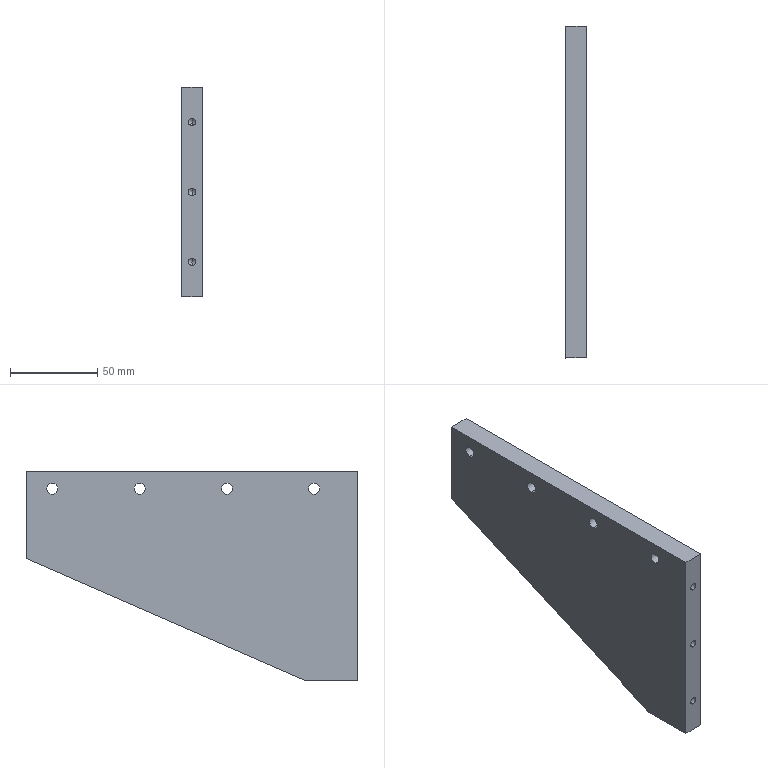Component | SolidWorks | V1ZHXTZ-AxisMountingPlateReinforcementPlateSB1-1 | 1 solid | 39 faces | box 12 x 190 x 120 mm | volume 202405 mm3 | cylinder 22 | plane 11 | cone 6 | commonest cylinder face diameters 11 x8 6.4 x8 4.2 x6
STEP:
#1=COLOUR_RGB('',0.7922,0.8196,0.9333);
#2=FILL_AREA_STYLE_COLOUR('',#1);
#3=FILL_AREA_STYLE('',(#2));
#4=SURFACE_STYLE_FILL_AREA(#3);
#5=SURFACE_SIDE_STYLE('',(#4));
#6=SURFACE_STYLE_USAGE(.BOTH.,#5);
#7=PRESENTATION_STYLE_ASSIGNMENT((#6));
#8=CARTESIAN_POINT('',(9.745,-12.863,21.687));
#9=VERTEX_POINT('',#8);
#10=CARTESIAN_POINT('',(9.745,-12.863,21.521));
#11=VERTEX_POINT('',#10);
#12=CARTESIAN_POINT('',(9.745,-12.863,21.604));
#13=DIRECTION('',(0.,-1.,-0.));
#14=DIRECTION('',(0.,0.,-1.));
#15=AXIS2_PLACEMENT_3D('',#12,#13,#14);
#16=CIRCLE('',#15,0.08268);
#17=EDGE_CURVE('',#9,#11,#16,.T.);
#18=ORIENTED_EDGE('',*,*,#17,.F.);
#19=CARTESIAN_POINT('',(9.745,-13.548,21.687));
#20=VERTEX_POINT('',#19);
#21=CARTESIAN_POINT('',(9.745,-13.548,21.687));
#22=DIRECTION('',(0.,-1.,-0.));
#23=VECTOR('',#22,39.37);
#24=LINE('',#21,#23);
#25=EDGE_CURVE('',#9,#20,#24,.T.);
#26=ORIENTED_EDGE('',*,*,#25,.T.);
#27=CARTESIAN_POINT('',(9.745,-13.548,21.521));
#28=VERTEX_POINT('',#27);
#29=CARTESIAN_POINT('',(9.745,-13.548,21.604));
#30=DIRECTION('',(0.,-1.,-0.));
#31=DIRECTION('',(0.,0.,-1.));
#32=AXIS2_PLACEMENT_3D('',#29,#30,#31);
#33=CIRCLE('',#32,0.08268);
#34=EDGE_CURVE('',#20,#28,#33,.T.);
#35=ORIENTED_EDGE('',*,*,#34,.T.);
#36=CARTESIAN_POINT('',(9.745,-13.548,21.521));
#37=DIRECTION('',(0.,-1.,-0.));
#38=VECTOR('',#37,39.37);
#39=LINE('',#36,#38);
#40=EDGE_CURVE('',#11,#28,#39,.T.);
#41=ORIENTED_EDGE('',*,*,#40,.F.);
#42=EDGE_LOOP('',(#18,#26,#35,#41));
#43=FACE_OUTER_BOUND('',#42,.T.);
#44=CARTESIAN_POINT('',(9.745,-13.548,21.604));
#45=DIRECTION('',(0.,-1.,-0.));
#46=DIRECTION('',(0.,0.,-1.));
#47=AXIS2_PLACEMENT_3D('',#44,#45,#46);
#48=CYLINDRICAL_SURFACE('',#47,0.08268);
#49=ADVANCED_FACE('',(#43),#48,.F.);
#50=CARTESIAN_POINT('',(9.745,-12.814,21.604));
#51=VERTEX_POINT('',#50);
#52=CARTESIAN_POINT('',(9.745,-12.863,21.521));
#53=DIRECTION('',(0.,-0.515,-0.8572));
#54=VECTOR('',#53,39.37);
#55=LINE('',#52,#54);
#56=EDGE_CURVE('',#51,#11,#55,.T.);
#57=ORIENTED_EDGE('',*,*,#56,.F.);
#58=CARTESIAN_POINT('',(9.745,-12.863,21.687));
#59=DIRECTION('',(0.,-0.515,0.8572));
#60=VECTOR('',#59,39.37);
#61=LINE('',#58,#60);
#62=EDGE_CURVE('',#51,#9,#61,.T.);
#63=ORIENTED_EDGE('',*,*,#62,.T.);
#64=ORIENTED_EDGE('',*,*,#17,.T.);
#65=EDGE_LOOP('',(#57,#63,#64));
#66=FACE_OUTER_BOUND('',#65,.T.);
#67=CARTESIAN_POINT('',(9.745,-12.863,21.604));
#68=DIRECTION('',(0.,-1.,-0.));
#69=DIRECTION('',(0.,0.,-1.));
#70=AXIS2_PLACEMENT_3D('',#67,#68,#69);
#71=CONICAL_SURFACE('',#70,0.08268,1.03);
#72=ADVANCED_FACE('',(#66),#71,.F.);
#73=CARTESIAN_POINT('',(9.745,-12.863,20.112));
#74=VERTEX_POINT('',#73);
#75=CARTESIAN_POINT('',(9.745,-12.863,19.946));
#76=VERTEX_POINT('',#75);
#77=CARTESIAN_POINT('',(9.745,-12.863,20.029));
#78=DIRECTION('',(0.,-1.,-0.));
#79=DIRECTION('',(0.,0.,-1.));
#80=AXIS2_PLACEMENT_3D('',#77,#78,#79);
#81=CIRCLE('',#80,0.08268);
#82=EDGE_CURVE('',#74,#76,#81,.T.);
#83=ORIENTED_EDGE('',*,*,#82,.F.);
#84=CARTESIAN_POINT('',(9.745,-13.548,20.112));
#85=VERTEX_POINT('',#84);
#86=CARTESIAN_POINT('',(9.745,-13.548,20.112));
#87=DIRECTION('',(0.,-1.,-0.));
#88=VECTOR('',#87,39.37);
#89=LINE('',#86,#88);
#90=EDGE_CURVE('',#74,#85,#89,.T.);
#91=ORIENTED_EDGE('',*,*,#90,.T.);
#92=CARTESIAN_POINT('',(9.745,-13.548,19.946));
#93=VERTEX_POINT('',#92);
#94=CARTESIAN_POINT('',(9.745,-13.548,20.029));
#95=DIRECTION('',(0.,-1.,-0.));
#96=DIRECTION('',(0.,0.,-1.));
#97=AXIS2_PLACEMENT_3D('',#94,#95,#96);
#98=CIRCLE('',#97,0.08268);
#99=EDGE_CURVE('',#85,#93,#98,.T.);
#100=ORIENTED_EDGE('',*,*,#99,.T.);
#101=CARTESIAN_POINT('',(9.745,-13.548,19.946));
#102=DIRECTION('',(0.,-1.,-0.));
#103=VECTOR('',#102,39.37);
#104=LINE('',#101,#103);
#105=EDGE_CURVE('',#76,#93,#104,.T.);
#106=ORIENTED_EDGE('',*,*,#105,.F.);
#107=EDGE_LOOP('',(#83,#91,#100,#106));
#108=FACE_OUTER_BOUND('',#107,.T.);
#109=CARTESIAN_POINT('',(9.745,-13.548,20.029));
#110=DIRECTION('',(0.,-1.,-0.));
#111=DIRECTION('',(0.,0.,-1.));
#112=AXIS2_PLACEMENT_3D('',#109,#110,#111);
#113=CYLINDRICAL_SURFACE('',#112,0.08268);
#114=ADVANCED_FACE('',(#108),#113,.F.);
#115=CARTESIAN_POINT('',(9.745,-12.814,20.029));
#116=VERTEX_POINT('',#115);
#117=CARTESIAN_POINT('',(9.745,-12.863,19.946));
#118=DIRECTION('',(0.,-0.515,-0.8572));
#119=VECTOR('',#118,39.37);
#120=LINE('',#117,#119);
#121=EDGE_CURVE('',#116,#76,#120,.T.);
#122=ORIENTED_EDGE('',*,*,#121,.F.);
#123=CARTESIAN_POINT('',(9.745,-12.863,20.112));
#124=DIRECTION('',(0.,-0.515,0.8572));
#125=VECTOR('',#124,39.37);
#126=LINE('',#123,#125);
#127=EDGE_CURVE('',#116,#74,#126,.T.);
#128=ORIENTED_EDGE('',*,*,#127,.T.);
#129=ORIENTED_EDGE('',*,*,#82,.T.);
#130=EDGE_LOOP('',(#122,#128,#129));
#131=FACE_OUTER_BOUND('',#130,.T.);
#132=CARTESIAN_POINT('',(9.745,-12.863,20.029));
#133=DIRECTION('',(0.,-1.,-0.));
#134=DIRECTION('',(0.,0.,-1.));
#135=AXIS2_PLACEMENT_3D('',#132,#133,#134);
#136=CONICAL_SURFACE('',#135,0.08268,1.03);
#137=ADVANCED_FACE('',(#131),#136,.F.);
#138=CARTESIAN_POINT('',(9.745,-12.863,18.537));
#139=VERTEX_POINT('',#138);
#140=CARTESIAN_POINT('',(9.745,-12.863,18.372));
#141=VERTEX_POINT('',#140);
#142=CARTESIAN_POINT('',(9.745,-12.863,18.454));
#143=DIRECTION('',(0.,-1.,-0.));
#144=DIRECTION('',(0.,0.,-1.));
#145=AXIS2_PLACEMENT_3D('',#142,#143,#144);
#146=CIRCLE('',#145,0.08268);
#147=EDGE_CURVE('',#139,#141,#146,.T.);
#148=ORIENTED_EDGE('',*,*,#147,.F.);
#149=CARTESIAN_POINT('',(9.745,-13.548,18.537));
#150=VERTEX_POINT('',#149);
#151=CARTESIAN_POINT('',(9.745,-13.548,18.537));
#152=DIRECTION('',(0.,-1.,-0.));
#153=VECTOR('',#152,39.37);
#154=LINE('',#151,#153);
#155=EDGE_CURVE('',#139,#150,#154,.T.);
#156=ORIENTED_EDGE('',*,*,#155,.T.);
#157=CARTESIAN_POINT('',(9.745,-13.548,18.372));
#158=VERTEX_POINT('',#157);
#159=CARTESIAN_POINT('',(9.745,-13.548,18.454));
#160=DIRECTION('',(0.,-1.,-0.));
#161=DIRECTION('',(0.,0.,-1.));
#162=AXIS2_PLACEMENT_3D('',#159,#160,#161);
#163=CIRCLE('',#162,0.08268);
#164=EDGE_CURVE('',#150,#158,#163,.T.);
#165=ORIENTED_EDGE('',*,*,#164,.T.);
#166=CARTESIAN_POINT('',(9.745,-13.548,18.372));
#167=DIRECTION('',(0.,-1.,-0.));
#168=VECTOR('',#167,39.37);
#169=LINE('',#166,#168);
#170=EDGE_CURVE('',#141,#158,#169,.T.);
#171=ORIENTED_EDGE('',*,*,#170,.F.);
#172=EDGE_LOOP('',(#148,#156,#165,#171));
#173=FACE_OUTER_BOUND('',#172,.T.);
#174=CARTESIAN_POINT('',(9.745,-13.548,18.454));
#175=DIRECTION('',(0.,-1.,-0.));
#176=DIRECTION('',(0.,0.,-1.));
#177=AXIS2_PLACEMENT_3D('',#174,#175,#176);
#178=CYLINDRICAL_SURFACE('',#177,0.08268);
#179=ADVANCED_FACE('',(#173),#178,.F.);
#180=CARTESIAN_POINT('',(9.745,-12.814,18.454));
#181=VERTEX_POINT('',#180);
#182=CARTESIAN_POINT('',(9.745,-12.863,18.372));
#183=DIRECTION('',(0.,-0.515,-0.8572));
#184=VECTOR('',#183,39.37);
#185=LINE('',#182,#184);
#186=EDGE_CURVE('',#181,#141,#185,.T.);
#187=ORIENTED_EDGE('',*,*,#186,.F.);
#188=CARTESIAN_POINT('',(9.745,-12.863,18.537));
#189=DIRECTION('',(0.,-0.515,0.8572));
#190=VECTOR('',#189,39.37);
#191=LINE('',#188,#190);
#192=EDGE_CURVE('',#181,#139,#191,.T.);
#193=ORIENTED_EDGE('',*,*,#192,.T.);
#194=ORIENTED_EDGE('',*,*,#147,.T.);
#195=EDGE_LOOP('',(#187,#193,#194));
#196=FACE_OUTER_BOUND('',#195,.T.);
#197=CARTESIAN_POINT('',(9.745,-12.863,18.454));
#198=DIRECTION('',(0.,-1.,-0.));
#199=DIRECTION('',(0.,0.,-1.));
#200=AXIS2_PLACEMENT_3D('',#197,#198,#199);
#201=CONICAL_SURFACE('',#200,0.08268,1.03);
#202=ADVANCED_FACE('',(#196),#201,.F.);
#203=CARTESIAN_POINT('',(9.713,-12.564,21.781));
#204=VERTEX_POINT('',#203);
#205=CARTESIAN_POINT('',(9.713,-12.564,22.214));
#206=VERTEX_POINT('',#205);
#207=CARTESIAN_POINT('',(9.713,-12.564,21.998));
#208=DIRECTION('',(1.,0.,-0.));
#209=DIRECTION('',(0.,-0.,1.));
#210=AXIS2_PLACEMENT_3D('',#207,#208,#209);
#211=CIRCLE('',#210,0.2165);
#212=EDGE_CURVE('',#204,#206,#211,.T.);
#213=ORIENTED_EDGE('',*,*,#212,.F.);
#214=CARTESIAN_POINT('',(9.981,-12.564,21.781));
#215=VERTEX_POINT('',#214);
#216=CARTESIAN_POINT('',(9.981,-12.564,21.781));
#217=DIRECTION('',(1.,0.,-0.));
#218=VECTOR('',#217,39.37);
#219=LINE('',#216,#218);
#220=EDGE_CURVE('',#204,#215,#219,.T.);
#221=ORIENTED_EDGE('',*,*,#220,.T.);
#222=CARTESIAN_POINT('',(9.981,-12.564,22.214));
#223=VERTEX_POINT('',#222);
#224=CARTESIAN_POINT('',(9.981,-12.564,21.998));
#225=DIRECTION('',(1.,0.,-0.));
#226=DIRECTION('',(0.,-0.,1.));
#227=AXIS2_PLACEMENT_3D('',#224,#225,#226);
#228=CIRCLE('',#227,0.2165);
#229=EDGE_CURVE('',#215,#223,#228,.T.);
#230=ORIENTED_EDGE('',*,*,#229,.T.);
#231=CARTESIAN_POINT('',(9.981,-12.564,22.214));
#232=DIRECTION('',(1.,0.,-0.));
#233=VECTOR('',#232,39.37);
#234=LINE('',#231,#233);
#235=EDGE_CURVE('',#206,#223,#234,.T.);
#236=ORIENTED_EDGE('',*,*,#235,.F.);
#237=EDGE_LOOP('',(#213,#221,#230,#236));
#238=FACE_OUTER_BOUND('',#237,.T.);
#239=CARTESIAN_POINT('',(9.981,-12.564,21.998));
#240=DIRECTION('',(1.,0.,-0.));
#241=DIRECTION('',(0.,-0.,1.));
#242=AXIS2_PLACEMENT_3D('',#239,#240,#241);
#243=CYLINDRICAL_SURFACE('',#242,0.2165);
#244=ADVANCED_FACE('',(#238),#243,.F.);
#245=CARTESIAN_POINT('',(9.509,-12.564,21.872));
#246=VERTEX_POINT('',#245);
#247=CARTESIAN_POINT('',(9.509,-12.564,22.124));
#248=VERTEX_POINT('',#247);
#249=CARTESIAN_POINT('',(9.509,-12.564,21.998));
#250=DIRECTION('',(1.,0.,-0.));
#251=DIRECTION('',(0.,-0.,1.));
#252=AXIS2_PLACEMENT_3D('',#249,#250,#251);
#253=CIRCLE('',#252,0.126);
#254=EDGE_CURVE('',#246,#248,#253,.T.);
#255=ORIENTED_EDGE('',*,*,#254,.F.);
#256=CARTESIAN_POINT('',(9.713,-12.564,21.872));
#257=VERTEX_POINT('',#256);
#258=CARTESIAN_POINT('',(9.981,-12.564,21.872));
#259=DIRECTION('',(1.,0.,-0.));
#260=VECTOR('',#259,39.37);
#261=LINE('',#258,#260);
#262=EDGE_CURVE('',#246,#257,#261,.T.);
#263=ORIENTED_EDGE('',*,*,#262,.T.);
#264=CARTESIAN_POINT('',(9.713,-12.564,22.124));
#265=VERTEX_POINT('',#264);
#266=CARTESIAN_POINT('',(9.713,-12.564,21.998));
#267=DIRECTION('',(1.,0.,-0.));
#268=DIRECTION('',(0.,-0.,1.));
#269=AXIS2_PLACEMENT_3D('',#266,#267,#268);
#270=CIRCLE('',#269,0.126);
#271=EDGE_CURVE('',#257,#265,#270,.T.);
#272=ORIENTED_EDGE('',*,*,#271,.T.);
#273=CARTESIAN_POINT('',(9.981,-12.564,22.124));
#274=DIRECTION('',(1.,0.,-0.));
#275=VECTOR('',#274,39.37);
#276=LINE('',#273,#275);
#277=EDGE_CURVE('',#248,#265,#276,.T.);
#278=ORIENTED_EDGE('',*,*,#277,.F.);
#279=EDGE_LOOP('',(#255,#263,#272,#278));
#280=FACE_OUTER_BOUND('',#279,.T.);
#281=CARTESIAN_POINT('',(9.981,-12.564,21.998));
#282=DIRECTION('',(1.,0.,-0.));
#283=DIRECTION('',(0.,-0.,1.));
#284=AXIS2_PLACEMENT_3D('',#281,#282,#283);
#285=CYLINDRICAL_SURFACE('',#284,0.126);
#286=ADVANCED_FACE('',(#280),#285,.F.);
#287=CARTESIAN_POINT('',(9.713,-10.596,21.781));
#288=VERTEX_POINT('',#287);
#289=CARTESIAN_POINT('',(9.713,-10.596,22.214));
#290=VERTEX_POINT('',#289);
#291=CARTESIAN_POINT('',(9.713,-10.596,21.998));
#292=DIRECTION('',(1.,0.,-0.));
#293=DIRECTION('',(0.,-0.,1.));
#294=AXIS2_PLACEMENT_3D('',#291,#292,#293);
#295=CIRCLE('',#294,0.2165);
#296=EDGE_CURVE('',#288,#290,#295,.T.);
#297=ORIENTED_EDGE('',*,*,#296,.F.);
#298=CARTESIAN_POINT('',(9.981,-10.596,21.781));
#299=VERTEX_POINT('',#298);
#300=CARTESIAN_POINT('',(9.981,-10.596,21.781));
#301=DIRECTION('',(1.,0.,-0.));
#302=VECTOR('',#301,39.37);
#303=LINE('',#300,#302);
#304=EDGE_CURVE('',#288,#299,#303,.T.);
#305=ORIENTED_EDGE('',*,*,#304,.T.);
#306=CARTESIAN_POINT('',(9.981,-10.596,22.214));
#307=VERTEX_POINT('',#306);
#308=CARTESIAN_POINT('',(9.981,-10.596,21.998));
#309=DIRECTION('',(1.,0.,-0.));
#310=DIRECTION('',(0.,-0.,1.));
#311=AXIS2_PLACEMENT_3D('',#308,#309,#310);
#312=CIRCLE('',#311,0.2165);
#313=EDGE_CURVE('',#299,#307,#312,.T.);
#314=ORIENTED_EDGE('',*,*,#313,.T.);
#315=CARTESIAN_POINT('',(9.981,-10.596,22.214));
#316=DIRECTION('',(1.,0.,-0.));
#317=VECTOR('',#316,39.37);
#318=LINE('',#315,#317);
#319=EDGE_CURVE('',#290,#307,#318,.T.);
#320=ORIENTED_EDGE('',*,*,#319,.F.);
#321=EDGE_LOOP('',(#297,#305,#314,#320));
#322=FACE_OUTER_BOUND('',#321,.T.);
#323=CARTESIAN_POINT('',(9.981,-10.596,21.998));
#324=DIRECTION('',(1.,0.,-0.));
#325=DIRECTION('',(0.,-0.,1.));
#326=AXIS2_PLACEMENT_3D('',#323,#324,#325);
#327=CYLINDRICAL_SURFACE('',#326,0.2165);
#328=ADVANCED_FACE('',(#322),#327,.F.);
#329=CARTESIAN_POINT('',(9.509,-10.596,21.872));
#330=VERTEX_POINT('',#329);
#331=CARTESIAN_POINT('',(9.509,-10.596,22.124));
#332=VERTEX_POINT('',#331);
#333=CARTESIAN_POINT('',(9.509,-10.596,21.998));
#334=DIRECTION('',(1.,0.,-0.));
#335=DIRECTION('',(0.,-0.,1.));
#336=AXIS2_PLACEMENT_3D('',#333,#334,#335);
#337=CIRCLE('',#336,0.126);
#338=EDGE_CURVE('',#330,#332,#337,.T.);
#339=ORIENTED_EDGE('',*,*,#338,.F.);
#340=CARTESIAN_POINT('',(9.713,-10.596,21.872));
#341=VERTEX_POINT('',#340);
#342=CARTESIAN_POINT('',(9.981,-10.596,21.872));
#343=DIRECTION('',(1.,0.,-0.));
#344=VECTOR('',#343,39.37);
#345=LINE('',#342,#344);
#346=EDGE_CURVE('',#330,#341,#345,.T.);
#347=ORIENTED_EDGE('',*,*,#346,.T.);
#348=CARTESIAN_POINT('',(9.713,-10.596,22.124));
#349=VERTEX_POINT('',#348);
#350=CARTESIAN_POINT('',(9.713,-10.596,21.998));
#351=DIRECTION('',(1.,0.,-0.));
#352=DIRECTION('',(0.,-0.,1.));
#353=AXIS2_PLACEMENT_3D('',#350,#351,#352);
#354=CIRCLE('',#353,0.126);
#355=EDGE_CURVE('',#341,#349,#354,.T.);
#356=ORIENTED_EDGE('',*,*,#355,.T.);
#357=CARTESIAN_POINT('',(9.981,-10.596,22.124));
#358=DIRECTION('',(1.,0.,-0.));
#359=VECTOR('',#358,39.37);
#360=LINE('',#357,#359);
#361=EDGE_CURVE('',#332,#349,#360,.T.);
#362=ORIENTED_EDGE('',*,*,#361,.F.);
#363=EDGE_LOOP('',(#339,#347,#356,#362));
#364=FACE_OUTER_BOUND('',#363,.T.);
#365=CARTESIAN_POINT('',(9.981,-10.596,21.998));
#366=DIRECTION('',(1.,0.,-0.));
#367=DIRECTION('',(0.,-0.,1.));
#368=AXIS2_PLACEMENT_3D('',#365,#366,#367);
#369=CYLINDRICAL_SURFACE('',#368,0.126);
#370=ADVANCED_FACE('',(#364),#369,.F.);
#371=CARTESIAN_POINT('',(9.713,-8.627,21.781));
#372=VERTEX_POINT('',#371);
#373=CARTESIAN_POINT('',(9.713,-8.627,22.214));
#374=VERTEX_POINT('',#373);
#375=CARTESIAN_POINT('',(9.713,-8.627,21.998));
#376=DIRECTION('',(1.,0.,-0.));
#377=DIRECTION('',(0.,-0.,1.));
#378=AXIS2_PLACEMENT_3D('',#375,#376,#377);
#379=CIRCLE('',#378,0.2165);
#380=EDGE_CURVE('',#372,#374,#379,.T.);
#381=ORIENTED_EDGE('',*,*,#380,.F.);
#382=CARTESIAN_POINT('',(9.981,-8.627,21.781));
#383=VERTEX_POINT('',#382);
#384=CARTESIAN_POINT('',(9.981,-8.627,21.781));
#385=DIRECTION('',(1.,0.,-0.));
#386=VECTOR('',#385,39.37);
#387=LINE('',#384,#386);
#388=EDGE_CURVE('',#372,#383,#387,.T.);
#389=ORIENTED_EDGE('',*,*,#388,.T.);
#390=CARTESIAN_POINT('',(9.981,-8.627,22.214));
#391=VERTEX_POINT('',#390);
#392=CARTESIAN_POINT('',(9.981,-8.627,21.998));
#393=DIRECTION('',(1.,0.,-0.));
#394=DIRECTION('',(0.,-0.,1.));
#395=AXIS2_PLACEMENT_3D('',#392,#393,#394);
#396=CIRCLE('',#395,0.2165);
#397=EDGE_CURVE('',#383,#391,#396,.T.);
#398=ORIENTED_EDGE('',*,*,#397,.T.);
#399=CARTESIAN_POINT('',(9.981,-8.627,22.214));
#400=DIRECTION('',(1.,0.,-0.));
#401=VECTOR('',#400,39.37);
#402=LINE('',#399,#401);
#403=EDGE_CURVE('',#374,#391,#402,.T.);
#404=ORIENTED_EDGE('',*,*,#403,.F.);
#405=EDGE_LOOP('',(#381,#389,#398,#404));
#406=FACE_OUTER_BOUND('',#405,.T.);
#407=CARTESIAN_POINT('',(9.981,-8.627,21.998));
#408=DIRECTION('',(1.,0.,-0.));
#409=DIRECTION('',(0.,-0.,1.));
#410=AXIS2_PLACEMENT_3D('',#407,#408,#409);
#411=CYLINDRICAL_SURFACE('',#410,0.2165);
#412=ADVANCED_FACE('',(#406),#411,.F.);
#413=CARTESIAN_POINT('',(9.509,-8.627,21.872));
#414=VERTEX_POINT('',#413);
#415=CARTESIAN_POINT('',(9.509,-8.627,22.124));
#416=VERTEX_POINT('',#415);
#417=CARTESIAN_POINT('',(9.509,-8.627,21.998));
#418=DIRECTION('',(1.,0.,-0.));
#419=DIRECTION('',(0.,-0.,1.));
#420=AXIS2_PLACEMENT_3D('',#417,#418,#419);
#421=CIRCLE('',#420,0.126);
#422=EDGE_CURVE('',#414,#416,#421,.T.);
#423=ORIENTED_EDGE('',*,*,#422,.F.);
#424=CARTESIAN_POINT('',(9.713,-8.627,21.872));
#425=VERTEX_POINT('',#424);
#426=CARTESIAN_POINT('',(9.981,-8.627,21.872));
#427=DIRECTION('',(1.,0.,-0.));
#428=VECTOR('',#427,39.37);
#429=LINE('',#426,#428);
#430=EDGE_CURVE('',#414,#425,#429,.T.);
#431=ORIENTED_EDGE('',*,*,#430,.T.);
#432=CARTESIAN_POINT('',(9.713,-8.627,22.124));
#433=VERTEX_POINT('',#432);
#434=CARTESIAN_POINT('',(9.713,-8.627,21.998));
#435=DIRECTION('',(1.,0.,-0.));
#436=DIRECTION('',(0.,-0.,1.));
#437=AXIS2_PLACEMENT_3D('',#434,#435,#436);
#438=CIRCLE('',#437,0.126);
#439=EDGE_CURVE('',#425,#433,#438,.T.);
#440=ORIENTED_EDGE('',*,*,#439,.T.);
#441=CARTESIAN_POINT('',(9.981,-8.627,22.124));
#442=DIRECTION('',(1.,0.,-0.));
#443=VECTOR('',#442,39.37);
#444=LINE('',#441,#443);
#445=EDGE_CURVE('',#416,#433,#444,.T.);
#446=ORIENTED_EDGE('',*,*,#445,.F.);
#447=EDGE_LOOP('',(#423,#431,#440,#446));
#448=FACE_OUTER_BOUND('',#447,.T.);
#449=CARTESIAN_POINT('',(9.981,-8.627,21.998));
#450=DIRECTION('',(1.,0.,-0.));
#451=DIRECTION('',(0.,-0.,1.));
#452=AXIS2_PLACEMENT_3D('',#449,#450,#451);
#453=CYLINDRICAL_SURFACE('',#452,0.126);
#454=ADVANCED_FACE('',(#448),#453,.F.);
#455=CARTESIAN_POINT('',(9.713,-6.659,21.781));
#456=VERTEX_POINT('',#455);
#457=CARTESIAN_POINT('',(9.713,-6.659,22.214));
#458=VERTEX_POINT('',#457);
#459=CARTESIAN_POINT('',(9.713,-6.659,21.998));
#460=DIRECTION('',(1.,0.,-0.));
#461=DIRECTION('',(0.,-0.,1.));
#462=AXIS2_PLACEMENT_3D('',#459,#460,#461);
#463=CIRCLE('',#462,0.2165);
#464=EDGE_CURVE('',#456,#458,#463,.T.);
#465=ORIENTED_EDGE('',*,*,#464,.F.);
#466=CARTESIAN_POINT('',(9.981,-6.659,21.781));
#467=VERTEX_POINT('',#466);
#468=CARTESIAN_POINT('',(9.981,-6.659,21.781));
#469=DIRECTION('',(1.,0.,-0.));
#470=VECTOR('',#469,39.37);
#471=LINE('',#468,#470);
#472=EDGE_CURVE('',#456,#467,#471,.T.);
#473=ORIENTED_EDGE('',*,*,#472,.T.);
#474=CARTESIAN_POINT('',(9.981,-6.659,22.214));
#475=VERTEX_POINT('',#474);
#476=CARTESIAN_POINT('',(9.981,-6.659,21.998));
#477=DIRECTION('',(1.,0.,-0.));
#478=DIRECTION('',(0.,-0.,1.));
#479=AXIS2_PLACEMENT_3D('',#476,#477,#478);
#480=CIRCLE('',#479,0.2165);
#481=EDGE_CURVE('',#467,#475,#480,.T.);
#482=ORIENTED_EDGE('',*,*,#481,.T.);
#483=CARTESIAN_POINT('',(9.981,-6.659,22.214));
#484=DIRECTION('',(1.,0.,-0.));
#485=VECTOR('',#484,39.37);
#486=LINE('',#483,#485);
#487=EDGE_CURVE('',#458,#475,#486,.T.);
#488=ORIENTED_EDGE('',*,*,#487,.F.);
#489=EDGE_LOOP('',(#465,#473,#482,#488));
#490=FACE_OUTER_BOUND('',#489,.T.);
#491=CARTESIAN_POINT('',(9.981,-6.659,21.998));
#492=DIRECTION('',(1.,0.,-0.));
#493=DIRECTION('',(0.,-0.,1.));
#494=AXIS2_PLACEMENT_3D('',#491,#492,#493);
#495=CYLINDRICAL_SURFACE('',#494,0.2165);
#496=ADVANCED_FACE('',(#490),#495,.F.);
#497=CARTESIAN_POINT('',(9.509,-6.659,21.872));
#498=VERTEX_POINT('',#497);
#499=CARTESIAN_POINT('',(9.509,-6.659,22.124));
#500=VERTEX_POINT('',#499);
#501=CARTESIAN_POINT('',(9.509,-6.659,21.998));
#502=DIRECTION('',(1.,0.,-0.));
#503=DIRECTION('',(0.,-0.,1.));
#504=AXIS2_PLACEMENT_3D('',#501,#502,#503);
#505=CIRCLE('',#504,0.126);
#506=EDGE_CURVE('',#498,#500,#505,.T.);
#507=ORIENTED_EDGE('',*,*,#506,.F.);
#508=CARTESIAN_POINT('',(9.713,-6.659,21.872));
#509=VERTEX_POINT('',#508);
#510=CARTESIAN_POINT('',(9.981,-6.659,21.872));
#511=DIRECTION('',(1.,0.,-0.));
#512=VECTOR('',#511,39.37);
#513=LINE('',#510,#512);
#514=EDGE_CURVE('',#498,#509,#513,.T.);
#515=ORIENTED_EDGE('',*,*,#514,.T.);
#516=CARTESIAN_POINT('',(9.713,-6.659,22.124));
#517=VERTEX_POINT('',#516);
#518=CARTESIAN_POINT('',(9.713,-6.659,21.998));
#519=DIRECTION('',(1.,0.,-0.));
#520=DIRECTION('',(0.,-0.,1.));
#521=AXIS2_PLACEMENT_3D('',#518,#519,#520);
#522=CIRCLE('',#521,0.126);
#523=EDGE_CURVE('',#509,#517,#522,.T.);
#524=ORIENTED_EDGE('',*,*,#523,.T.);
#525=CARTESIAN_POINT('',(9.981,-6.659,22.124));
#526=DIRECTION('',(1.,0.,-0.));
#527=VECTOR('',#526,39.37);
#528=LINE('',#525,#527);
#529=EDGE_CURVE('',#500,#517,#528,.T.);
#530=ORIENTED_EDGE('',*,*,#529,.F.);
#531=EDGE_LOOP('',(#507,#515,#524,#530));
#532=FACE_OUTER_BOUND('',#531,.T.);
#533=CARTESIAN_POINT('',(9.981,-6.659,21.998));
#534=DIRECTION('',(1.,0.,-0.));
#535=DIRECTION('',(0.,-0.,1.));
#536=AXIS2_PLACEMENT_3D('',#533,#534,#535);
#537=CYLINDRICAL_SURFACE('',#536,0.126);
#538=ADVANCED_FACE('',(#532),#537,.F.);
#539=CARTESIAN_POINT('',(9.745,-13.548,21.604));
#540=DIRECTION('',(0.,-1.,-0.));
#541=DIRECTION('',(0.,0.,-1.));
#542=AXIS2_PLACEMENT_3D('',#539,#540,#541);
#543=CIRCLE('',#542,0.08268);
#544=EDGE_CURVE('',#28,#20,#543,.T.);
#545=ORIENTED_EDGE('',*,*,#544,.F.);
#546=ORIENTED_EDGE('',*,*,#34,.F.);
#547=EDGE_LOOP('',(#545,#546));
#548=FACE_BOUND('',#547,.T.);
#549=CARTESIAN_POINT('',(9.745,-13.548,20.029));
#550=DIRECTION('',(0.,-1.,-0.));
#551=DIRECTION('',(0.,0.,-1.));
#552=AXIS2_PLACEMENT_3D('',#549,#550,#551);
#553=CIRCLE('',#552,0.08268);
#554=EDGE_CURVE('',#93,#85,#553,.T.);
#555=ORIENTED_EDGE('',*,*,#554,.F.);
#556=ORIENTED_EDGE('',*,*,#99,.F.);
#557=EDGE_LOOP('',(#555,#556));
#558=FACE_BOUND('',#557,.T.);
#559=CARTESIAN_POINT('',(9.745,-13.548,18.454));
#560=DIRECTION('',(0.,-1.,-0.));
#561=DIRECTION('',(0.,0.,-1.));
#562=AXIS2_PLACEMENT_3D('',#559,#560,#561);
#563=CIRCLE('',#562,0.08268);
#564=EDGE_CURVE('',#158,#150,#563,.T.);
#565=ORIENTED_EDGE('',*,*,#564,.F.);
#566=ORIENTED_EDGE('',*,*,#164,.F.);
#567=EDGE_LOOP('',(#565,#566));
#568=FACE_BOUND('',#567,.T.);
#569=CARTESIAN_POINT('',(9.509,-13.548,22.391));
#570=VERTEX_POINT('',#569);
#571=CARTESIAN_POINT('',(9.509,-13.548,17.667));
#572=VERTEX_POINT('',#571);
#573=CARTESIAN_POINT('',(9.509,-13.548,22.391));
#574=DIRECTION('',(-0.,0.,-1.));
#575=VECTOR('',#574,39.37);
#576=LINE('',#573,#575);
#577=EDGE_CURVE('',#570,#572,#576,.T.);
#578=ORIENTED_EDGE('',*,*,#577,.T.);
#579=CARTESIAN_POINT('',(9.981,-13.548,17.667));
#580=VERTEX_POINT('',#579);
#581=CARTESIAN_POINT('',(9.981,-13.548,17.667));
#582=DIRECTION('',(-1.,-0.,0.));
#583=VECTOR('',#582,39.37);
#584=LINE('',#581,#583);
#585=EDGE_CURVE('',#580,#572,#584,.T.);
#586=ORIENTED_EDGE('',*,*,#585,.F.);
#587=CARTESIAN_POINT('',(9.981,-13.548,22.391));
#588=VERTEX_POINT('',#587);
#589=CARTESIAN_POINT('',(9.981,-13.548,22.391));
#590=DIRECTION('',(-0.,0.,-1.));
#591=VECTOR('',#590,39.37);
#592=LINE('',#589,#591);
#593=EDGE_CURVE('',#588,#580,#592,.T.);
#594=ORIENTED_EDGE('',*,*,#593,.F.);
#595=CARTESIAN_POINT('',(9.981,-13.548,22.391));
#596=DIRECTION('',(-1.,-0.,0.));
#597=VECTOR('',#596,39.37);
#598=LINE('',#595,#597);
#599=EDGE_CURVE('',#588,#570,#598,.T.);
#600=ORIENTED_EDGE('',*,*,#599,.T.);
#601=EDGE_LOOP('',(#578,#586,#594,#600));
#602=FACE_OUTER_BOUND('',#601,.T.);
#603=CARTESIAN_POINT('',(9.981,-13.548,22.391));
#604=DIRECTION('',(-0.,1.,0.));
#605=DIRECTION('',(0.,-0.,1.));
#606=AXIS2_PLACEMENT_3D('',#603,#604,#605);
#607=PLANE('',#606);
#608=ADVANCED_FACE('',(#548,#558,#568,#602),#607,.F.);
#609=CARTESIAN_POINT('',(9.509,-12.367,17.667));
#610=VERTEX_POINT('',#609);
#611=CARTESIAN_POINT('',(9.509,-6.068,17.667));
#612=DIRECTION('',(-0.,1.,0.));
#613=VECTOR('',#612,39.37);
#614=LINE('',#611,#613);
#615=EDGE_CURVE('',#572,#610,#614,.T.);
#616=ORIENTED_EDGE('',*,*,#615,.T.);
#617=CARTESIAN_POINT('',(9.981,-12.367,17.667));
#618=VERTEX_POINT('',#617);
#619=CARTESIAN_POINT('',(9.981,-12.367,17.667));
#620=DIRECTION('',(1.,0.,-0.));
#621=VECTOR('',#620,39.37);
#622=LINE('',#619,#621);
#623=EDGE_CURVE('',#610,#618,#622,.T.);
#624=ORIENTED_EDGE('',*,*,#623,.T.);
#625=CARTESIAN_POINT('',(9.981,-6.068,17.667));
#626=DIRECTION('',(-0.,1.,0.));
#627=VECTOR('',#626,39.37);
#628=LINE('',#625,#627);
#629=EDGE_CURVE('',#580,#618,#628,.T.);
#630=ORIENTED_EDGE('',*,*,#629,.F.);
#631=ORIENTED_EDGE('',*,*,#585,.T.);
#632=EDGE_LOOP('',(#616,#624,#630,#631));
#633=FACE_OUTER_BOUND('',#632,.T.);
#634=CARTESIAN_POINT('',(9.981,-6.068,17.667));
#635=DIRECTION('',(0.,-0.,1.));
#636=DIRECTION('',(0.,-1.,-0.));
#637=AXIS2_PLACEMENT_3D('',#634,#635,#636);
#638=PLANE('',#637);
#639=ADVANCED_FACE('',(#633),#638,.F.);
#640=CARTESIAN_POINT('',(9.981,-6.068,20.423));
#641=VERTEX_POINT('',#640);
#642=CARTESIAN_POINT('',(9.981,-6.068,22.391));
#643=VERTEX_POINT('',#642);
#644=CARTESIAN_POINT('',(9.981,-6.068,22.391));
#645=DIRECTION('',(0.,-0.,1.));
#646=VECTOR('',#645,39.37);
#647=LINE('',#644,#646);
#648=EDGE_CURVE('',#641,#643,#647,.T.);
#649=ORIENTED_EDGE('',*,*,#648,.F.);
#650=CARTESIAN_POINT('',(9.509,-6.068,20.423));
#651=VERTEX_POINT('',#650);
#652=CARTESIAN_POINT('',(9.981,-6.068,20.423));
#653=DIRECTION('',(-1.,-0.,0.));
#654=VECTOR('',#653,39.37);
#655=LINE('',#652,#654);
#656=EDGE_CURVE('',#641,#651,#655,.T.);
#657=ORIENTED_EDGE('',*,*,#656,.T.);
#658=CARTESIAN_POINT('',(9.509,-6.068,22.391));
#659=VERTEX_POINT('',#658);
#660=CARTESIAN_POINT('',(9.509,-6.068,22.391));
#661=DIRECTION('',(0.,-0.,1.));
#662=VECTOR('',#661,39.37);
#663=LINE('',#660,#662);
#664=EDGE_CURVE('',#651,#659,#663,.T.);
#665=ORIENTED_EDGE('',*,*,#664,.T.);
#666=CARTESIAN_POINT('',(9.981,-6.068,22.391));
#667=DIRECTION('',(-1.,-0.,0.));
#668=VECTOR('',#667,39.37);
#669=LINE('',#666,#668);
#670=EDGE_CURVE('',#643,#659,#669,.T.);
#671=ORIENTED_EDGE('',*,*,#670,.F.);
#672=EDGE_LOOP('',(#649,#657,#665,#671));
#673=FACE_OUTER_BOUND('',#672,.T.);
#674=CARTESIAN_POINT('',(9.981,-6.068,22.391));
#675=DIRECTION('',(0.,-1.,-0.));
#676=DIRECTION('',(-0.,0.,-1.));
#677=AXIS2_PLACEMENT_3D('',#674,#675,#676);
#678=PLANE('',#677);
#679=ADVANCED_FACE('',(#673),#678,.F.);
#680=CARTESIAN_POINT('',(9.509,-6.068,22.391));
#681=DIRECTION('',(0.,-1.,-0.));
#682=VECTOR('',#681,39.37);
#683=LINE('',#680,#682);
#684=EDGE_CURVE('',#659,#570,#683,.T.);
#685=ORIENTED_EDGE('',*,*,#684,.T.);
#686=ORIENTED_EDGE('',*,*,#599,.F.);
#687=CARTESIAN_POINT('',(9.981,-6.068,22.391));
#688=DIRECTION('',(0.,-1.,-0.));
#689=VECTOR('',#688,39.37);
#690=LINE('',#687,#689);
#691=EDGE_CURVE('',#643,#588,#690,.T.);
#692=ORIENTED_EDGE('',*,*,#691,.F.);
#693=ORIENTED_EDGE('',*,*,#670,.T.);
#694=EDGE_LOOP('',(#685,#686,#692,#693));
#695=FACE_OUTER_BOUND('',#694,.T.);
#696=CARTESIAN_POINT('',(9.981,-6.068,22.391));
#697=DIRECTION('',(-0.,0.,-1.));
#698=DIRECTION('',(-0.,1.,0.));
#699=AXIS2_PLACEMENT_3D('',#696,#697,#698);
#700=PLANE('',#699);
#701=ADVANCED_FACE('',(#695),#700,.F.);
#702=CARTESIAN_POINT('',(9.981,-12.564,21.998));
#703=DIRECTION('',(1.,0.,-0.));
#704=DIRECTION('',(0.,-0.,1.));
#705=AXIS2_PLACEMENT_3D('',#702,#703,#704);
#706=CIRCLE('',#705,0.2165);
#707=EDGE_CURVE('',#223,#215,#706,.T.);
#708=ORIENTED_EDGE('',*,*,#707,.F.);
#709=ORIENTED_EDGE('',*,*,#229,.F.);
#710=EDGE_LOOP('',(#708,#709));
#711=FACE_BOUND('',#710,.T.);
#712=CARTESIAN_POINT('',(9.981,-10.596,21.998));
#713=DIRECTION('',(1.,0.,-0.));
#714=DIRECTION('',(0.,-0.,1.));
#715=AXIS2_PLACEMENT_3D('',#712,#713,#714);
#716=CIRCLE('',#715,0.2165);
#717=EDGE_CURVE('',#307,#299,#716,.T.);
#718=ORIENTED_EDGE('',*,*,#717,.F.);
#719=ORIENTED_EDGE('',*,*,#313,.F.);
#720=EDGE_LOOP('',(#718,#719));
#721=FACE_BOUND('',#720,.T.);
#722=CARTESIAN_POINT('',(9.981,-8.627,21.998));
#723=DIRECTION('',(1.,0.,-0.));
#724=DIRECTION('',(0.,-0.,1.));
#725=AXIS2_PLACEMENT_3D('',#722,#723,#724);
#726=CIRCLE('',#725,0.2165);
#727=EDGE_CURVE('',#391,#383,#726,.T.);
#728=ORIENTED_EDGE('',*,*,#727,.F.);
#729=ORIENTED_EDGE('',*,*,#397,.F.);
#730=EDGE_LOOP('',(#728,#729));
#731=FACE_BOUND('',#730,.T.);
#732=CARTESIAN_POINT('',(9.981,-6.659,21.998));
#733=DIRECTION('',(1.,0.,-0.));
#734=DIRECTION('',(0.,-0.,1.));
#735=AXIS2_PLACEMENT_3D('',#732,#733,#734);
#736=CIRCLE('',#735,0.2165);
#737=EDGE_CURVE('',#475,#467,#736,.T.);
#738=ORIENTED_EDGE('',*,*,#737,.F.);
#739=ORIENTED_EDGE('',*,*,#481,.F.);
#740=EDGE_LOOP('',(#738,#739));
#741=FACE_BOUND('',#740,.T.);
#742=ORIENTED_EDGE('',*,*,#629,.T.);
#743=CARTESIAN_POINT('',(9.981,-6.068,20.423));
#744=DIRECTION('',(-0.,0.9162,0.4008));
#745=VECTOR('',#744,39.37);
#746=LINE('',#743,#745);
#747=EDGE_CURVE('',#618,#641,#746,.T.);
#748=ORIENTED_EDGE('',*,*,#747,.T.);
#749=ORIENTED_EDGE('',*,*,#648,.T.);
#750=ORIENTED_EDGE('',*,*,#691,.T.);
#751=ORIENTED_EDGE('',*,*,#593,.T.);
#752=EDGE_LOOP('',(#742,#748,#749,#750,#751));
#753=FACE_OUTER_BOUND('',#752,.T.);
#754=CARTESIAN_POINT('',(9.981,-9.808,20.029));
#755=DIRECTION('',(-1.,-0.,0.));
#756=DIRECTION('',(-0.,0.,-1.));
#757=AXIS2_PLACEMENT_3D('',#754,#755,#756);
#758=PLANE('',#757);
#759=ADVANCED_FACE('',(#711,#721,#731,#741,#753),#758,.F.);
#760=CARTESIAN_POINT('',(9.509,-12.564,21.998));
#761=DIRECTION('',(1.,0.,-0.));
#762=DIRECTION('',(0.,-0.,1.));
#763=AXIS2_PLACEMENT_3D('',#760,#761,#762);
#764=CIRCLE('',#763,0.126);
#765=EDGE_CURVE('',#248,#246,#764,.T.);
#766=ORIENTED_EDGE('',*,*,#765,.T.);
#767=ORIENTED_EDGE('',*,*,#254,.T.);
#768=EDGE_LOOP('',(#766,#767));
#769=FACE_BOUND('',#768,.T.);
#770=CARTESIAN_POINT('',(9.509,-10.596,21.998));
#771=DIRECTION('',(1.,0.,-0.));
#772=DIRECTION('',(0.,-0.,1.));
#773=AXIS2_PLACEMENT_3D('',#770,#771,#772);
#774=CIRCLE('',#773,0.126);
#775=EDGE_CURVE('',#332,#330,#774,.T.);
#776=ORIENTED_EDGE('',*,*,#775,.T.);
#777=ORIENTED_EDGE('',*,*,#338,.T.);
#778=EDGE_LOOP('',(#776,#777));
#779=FACE_BOUND('',#778,.T.);
#780=CARTESIAN_POINT('',(9.509,-8.627,21.998));
#781=DIRECTION('',(1.,0.,-0.));
#782=DIRECTION('',(0.,-0.,1.));
#783=AXIS2_PLACEMENT_3D('',#780,#781,#782);
#784=CIRCLE('',#783,0.126);
#785=EDGE_CURVE('',#416,#414,#784,.T.);
#786=ORIENTED_EDGE('',*,*,#785,.T.);
#787=ORIENTED_EDGE('',*,*,#422,.T.);
#788=EDGE_LOOP('',(#786,#787));
#789=FACE_BOUND('',#788,.T.);
#790=CARTESIAN_POINT('',(9.509,-6.659,21.998));
#791=DIRECTION('',(1.,0.,-0.));
#792=DIRECTION('',(0.,-0.,1.));
#793=AXIS2_PLACEMENT_3D('',#790,#791,#792);
#794=CIRCLE('',#793,0.126);
#795=EDGE_CURVE('',#500,#498,#794,.T.);
#796=ORIENTED_EDGE('',*,*,#795,.T.);
#797=ORIENTED_EDGE('',*,*,#506,.T.);
#798=EDGE_LOOP('',(#796,#797));
#799=FACE_BOUND('',#798,.T.);
#800=ORIENTED_EDGE('',*,*,#664,.F.);
#801=CARTESIAN_POINT('',(9.509,-9.352,18.986));
#802=DIRECTION('',(0.,-0.9162,-0.4008));
#803=VECTOR('',#802,39.37);
#804=LINE('',#801,#803);
#805=EDGE_CURVE('',#651,#610,#804,.T.);
#806=ORIENTED_EDGE('',*,*,#805,.T.);
#807=ORIENTED_EDGE('',*,*,#615,.F.);
#808=ORIENTED_EDGE('',*,*,#577,.F.);
#809=ORIENTED_EDGE('',*,*,#684,.F.);
#810=EDGE_LOOP('',(#800,#806,#807,#808,#809));
#811=FACE_OUTER_BOUND('',#810,.T.);
#812=CARTESIAN_POINT('',(9.509,-9.808,20.029));
#813=DIRECTION('',(-1.,-0.,0.));
#814=DIRECTION('',(-0.,0.,-1.));
#815=AXIS2_PLACEMENT_3D('',#812,#813,#814);
#816=PLANE('',#815);
#817=ADVANCED_FACE('',(#769,#779,#789,#799,#811),#816,.T.);
#818=ORIENTED_EDGE('',*,*,#747,.F.);
#819=ORIENTED_EDGE('',*,*,#623,.F.);
#820=ORIENTED_EDGE('',*,*,#805,.F.);
#821=ORIENTED_EDGE('',*,*,#656,.F.);
#822=EDGE_LOOP('',(#818,#819,#820,#821));
#823=FACE_OUTER_BOUND('',#822,.T.);
#824=CARTESIAN_POINT('',(9.981,-6.068,20.423));
#825=DIRECTION('',(0.,-0.4008,0.9162));
#826=DIRECTION('',(-1.,-0.,0.));
#827=AXIS2_PLACEMENT_3D('',#824,#825,#826);
#828=PLANE('',#827);
#829=ADVANCED_FACE('',(#823),#828,.F.);
#830=ORIENTED_EDGE('',*,*,#514,.F.);
#831=ORIENTED_EDGE('',*,*,#795,.F.);
#832=ORIENTED_EDGE('',*,*,#529,.T.);
#833=CARTESIAN_POINT('',(9.713,-6.659,21.998));
#834=DIRECTION('',(1.,0.,-0.));
#835=DIRECTION('',(0.,-0.,1.));
#836=AXIS2_PLACEMENT_3D('',#833,#834,#835);
#837=CIRCLE('',#836,0.126);
#838=EDGE_CURVE('',#517,#509,#837,.T.);
#839=ORIENTED_EDGE('',*,*,#838,.T.);
#840=EDGE_LOOP('',(#830,#831,#832,#839));
#841=FACE_OUTER_BOUND('',#840,.T.);
#842=CARTESIAN_POINT('',(9.981,-6.659,21.998));
#843=DIRECTION('',(1.,0.,-0.));
#844=DIRECTION('',(0.,-0.,1.));
#845=AXIS2_PLACEMENT_3D('',#842,#843,#844);
#846=CYLINDRICAL_SURFACE('',#845,0.126);
#847=ADVANCED_FACE('',(#841),#846,.F.);
#848=ORIENTED_EDGE('',*,*,#838,.F.);
#849=ORIENTED_EDGE('',*,*,#523,.F.);
#850=EDGE_LOOP('',(#848,#849));
#851=FACE_BOUND('',#850,.T.);
#852=CARTESIAN_POINT('',(9.713,-6.659,21.998));
#853=DIRECTION('',(1.,0.,-0.));
#854=DIRECTION('',(0.,-0.,1.));
#855=AXIS2_PLACEMENT_3D('',#852,#853,#854);
#856=CIRCLE('',#855,0.2165);
#857=EDGE_CURVE('',#458,#456,#856,.T.);
#858=ORIENTED_EDGE('',*,*,#857,.T.);
#859=ORIENTED_EDGE('',*,*,#464,.T.);
#860=EDGE_LOOP('',(#858,#859));
#861=FACE_OUTER_BOUND('',#860,.T.);
#862=CARTESIAN_POINT('',(9.713,-6.785,21.998));
#863=DIRECTION('',(-1.,-0.,0.));
#864=DIRECTION('',(-0.,0.,-1.));
#865=AXIS2_PLACEMENT_3D('',#862,#863,#864);
#866=PLANE('',#865);
#867=ADVANCED_FACE('',(#851,#861),#866,.F.);
#868=ORIENTED_EDGE('',*,*,#472,.F.);
#869=ORIENTED_EDGE('',*,*,#857,.F.);
#870=ORIENTED_EDGE('',*,*,#487,.T.);
#871=ORIENTED_EDGE('',*,*,#737,.T.);
#872=EDGE_LOOP('',(#868,#869,#870,#871));
#873=FACE_OUTER_BOUND('',#872,.T.);
#874=CARTESIAN_POINT('',(9.981,-6.659,21.998));
#875=DIRECTION('',(1.,0.,-0.));
#876=DIRECTION('',(0.,-0.,1.));
#877=AXIS2_PLACEMENT_3D('',#874,#875,#876);
#878=CYLINDRICAL_SURFACE('',#877,0.2165);
#879=ADVANCED_FACE('',(#873),#878,.F.);
#880=ORIENTED_EDGE('',*,*,#430,.F.);
#881=ORIENTED_EDGE('',*,*,#785,.F.);
#882=ORIENTED_EDGE('',*,*,#445,.T.);
#883=CARTESIAN_POINT('',(9.713,-8.627,21.998));
#884=DIRECTION('',(1.,0.,-0.));
#885=DIRECTION('',(0.,-0.,1.));
#886=AXIS2_PLACEMENT_3D('',#883,#884,#885);
#887=CIRCLE('',#886,0.126);
#888=EDGE_CURVE('',#433,#425,#887,.T.);
#889=ORIENTED_EDGE('',*,*,#888,.T.);
#890=EDGE_LOOP('',(#880,#881,#882,#889));
#891=FACE_OUTER_BOUND('',#890,.T.);
#892=CARTESIAN_POINT('',(9.981,-8.627,21.998));
#893=DIRECTION('',(1.,0.,-0.));
#894=DIRECTION('',(0.,-0.,1.));
#895=AXIS2_PLACEMENT_3D('',#892,#893,#894);
#896=CYLINDRICAL_SURFACE('',#895,0.126);
#897=ADVANCED_FACE('',(#891),#896,.F.);
#898=ORIENTED_EDGE('',*,*,#888,.F.);
#899=ORIENTED_EDGE('',*,*,#439,.F.);
#900=EDGE_LOOP('',(#898,#899));
#901=FACE_BOUND('',#900,.T.);
#902=CARTESIAN_POINT('',(9.713,-8.627,21.998));
#903=DIRECTION('',(1.,0.,-0.));
#904=DIRECTION('',(0.,-0.,1.));
#905=AXIS2_PLACEMENT_3D('',#902,#903,#904);
#906=CIRCLE('',#905,0.2165);
#907=EDGE_CURVE('',#374,#372,#906,.T.);
#908=ORIENTED_EDGE('',*,*,#907,.T.);
#909=ORIENTED_EDGE('',*,*,#380,.T.);
#910=EDGE_LOOP('',(#908,#909));
#911=FACE_OUTER_BOUND('',#910,.T.);
#912=CARTESIAN_POINT('',(9.713,-8.753,21.998));
#913=DIRECTION('',(-1.,-0.,0.));
#914=DIRECTION('',(-0.,0.,-1.));
#915=AXIS2_PLACEMENT_3D('',#912,#913,#914);
#916=PLANE('',#915);
#917=ADVANCED_FACE('',(#901,#911),#916,.F.);
#918=ORIENTED_EDGE('',*,*,#388,.F.);
#919=ORIENTED_EDGE('',*,*,#907,.F.);
#920=ORIENTED_EDGE('',*,*,#403,.T.);
#921=ORIENTED_EDGE('',*,*,#727,.T.);
#922=EDGE_LOOP('',(#918,#919,#920,#921));
#923=FACE_OUTER_BOUND('',#922,.T.);
#924=CARTESIAN_POINT('',(9.981,-8.627,21.998));
#925=DIRECTION('',(1.,0.,-0.));
#926=DIRECTION('',(0.,-0.,1.));
#927=AXIS2_PLACEMENT_3D('',#924,#925,#926);
#928=CYLINDRICAL_SURFACE('',#927,0.2165);
#929=ADVANCED_FACE('',(#923),#928,.F.);
#930=ORIENTED_EDGE('',*,*,#346,.F.);
#931=ORIENTED_EDGE('',*,*,#775,.F.);
#932=ORIENTED_EDGE('',*,*,#361,.T.);
#933=CARTESIAN_POINT('',(9.713,-10.596,21.998));
#934=DIRECTION('',(1.,0.,-0.));
#935=DIRECTION('',(0.,-0.,1.));
#936=AXIS2_PLACEMENT_3D('',#933,#934,#935);
#937=CIRCLE('',#936,0.126);
#938=EDGE_CURVE('',#349,#341,#937,.T.);
#939=ORIENTED_EDGE('',*,*,#938,.T.);
#940=EDGE_LOOP('',(#930,#931,#932,#939));
#941=FACE_OUTER_BOUND('',#940,.T.);
#942=CARTESIAN_POINT('',(9.981,-10.596,21.998));
#943=DIRECTION('',(1.,0.,-0.));
#944=DIRECTION('',(0.,-0.,1.));
#945=AXIS2_PLACEMENT_3D('',#942,#943,#944);
#946=CYLINDRICAL_SURFACE('',#945,0.126);
#947=ADVANCED_FACE('',(#941),#946,.F.);
#948=ORIENTED_EDGE('',*,*,#938,.F.);
#949=ORIENTED_EDGE('',*,*,#355,.F.);
#950=EDGE_LOOP('',(#948,#949));
#951=FACE_BOUND('',#950,.T.);
#952=CARTESIAN_POINT('',(9.713,-10.596,21.998));
#953=DIRECTION('',(1.,0.,-0.));
#954=DIRECTION('',(0.,-0.,1.));
#955=AXIS2_PLACEMENT_3D('',#952,#953,#954);
#956=CIRCLE('',#955,0.2165);
#957=EDGE_CURVE('',#290,#288,#956,.T.);
#958=ORIENTED_EDGE('',*,*,#957,.T.);
#959=ORIENTED_EDGE('',*,*,#296,.T.);
#960=EDGE_LOOP('',(#958,#959));
#961=FACE_OUTER_BOUND('',#960,.T.);
#962=CARTESIAN_POINT('',(9.713,-10.722,21.998));
#963=DIRECTION('',(-1.,-0.,0.));
#964=DIRECTION('',(-0.,0.,-1.));
#965=AXIS2_PLACEMENT_3D('',#962,#963,#964);
#966=PLANE('',#965);
#967=ADVANCED_FACE('',(#951,#961),#966,.F.);
#968=ORIENTED_EDGE('',*,*,#304,.F.);
#969=ORIENTED_EDGE('',*,*,#957,.F.);
#970=ORIENTED_EDGE('',*,*,#319,.T.);
#971=ORIENTED_EDGE('',*,*,#717,.T.);
#972=EDGE_LOOP('',(#968,#969,#970,#971));
#973=FACE_OUTER_BOUND('',#972,.T.);
#974=CARTESIAN_POINT('',(9.981,-10.596,21.998));
#975=DIRECTION('',(1.,0.,-0.));
#976=DIRECTION('',(0.,-0.,1.));
#977=AXIS2_PLACEMENT_3D('',#974,#975,#976);
#978=CYLINDRICAL_SURFACE('',#977,0.2165);
#979=ADVANCED_FACE('',(#973),#978,.F.);
#980=ORIENTED_EDGE('',*,*,#262,.F.);
#981=ORIENTED_EDGE('',*,*,#765,.F.);
#982=ORIENTED_EDGE('',*,*,#277,.T.);
#983=CARTESIAN_POINT('',(9.713,-12.564,21.998));
#984=DIRECTION('',(1.,0.,-0.));
#985=DIRECTION('',(0.,-0.,1.));
#986=AXIS2_PLACEMENT_3D('',#983,#984,#985);
#987=CIRCLE('',#986,0.126);
#988=EDGE_CURVE('',#265,#257,#987,.T.);
#989=ORIENTED_EDGE('',*,*,#988,.T.);
#990=EDGE_LOOP('',(#980,#981,#982,#989));
#991=FACE_OUTER_BOUND('',#990,.T.);
#992=CARTESIAN_POINT('',(9.981,-12.564,21.998));
#993=DIRECTION('',(1.,0.,-0.));
#994=DIRECTION('',(0.,-0.,1.));
#995=AXIS2_PLACEMENT_3D('',#992,#993,#994);
#996=CYLINDRICAL_SURFACE('',#995,0.126);
#997=ADVANCED_FACE('',(#991),#996,.F.);
#998=ORIENTED_EDGE('',*,*,#988,.F.);
#999=ORIENTED_EDGE('',*,*,#271,.F.);
#1000=EDGE_LOOP('',(#998,#999));
#1001=FACE_BOUND('',#1000,.T.);
#1002=CARTESIAN_POINT('',(9.713,-12.564,21.998));
#1003=DIRECTION('',(1.,0.,-0.));
#1004=DIRECTION('',(0.,-0.,1.));
#1005=AXIS2_PLACEMENT_3D('',#1002,#1003,#1004);
#1006=CIRCLE('',#1005,0.2165);
#1007=EDGE_CURVE('',#206,#204,#1006,.T.);
#1008=ORIENTED_EDGE('',*,*,#1007,.T.);
#1009=ORIENTED_EDGE('',*,*,#212,.T.);
#1010=EDGE_LOOP('',(#1008,#1009));
#1011=FACE_OUTER_BOUND('',#1010,.T.);
#1012=CARTESIAN_POINT('',(9.713,-12.69,21.998));
#1013=DIRECTION('',(-1.,-0.,0.));
#1014=DIRECTION('',(-0.,0.,-1.));
#1015=AXIS2_PLACEMENT_3D('',#1012,#1013,#1014);
#1016=PLANE('',#1015);
#1017=ADVANCED_FACE('',(#1001,#1011),#1016,.F.);
#1018=ORIENTED_EDGE('',*,*,#220,.F.);
#1019=ORIENTED_EDGE('',*,*,#1007,.F.);
#1020=ORIENTED_EDGE('',*,*,#235,.T.);
#1021=ORIENTED_EDGE('',*,*,#707,.T.);
#1022=EDGE_LOOP('',(#1018,#1019,#1020,#1021));
#1023=FACE_OUTER_BOUND('',#1022,.T.);
#1024=CARTESIAN_POINT('',(9.981,-12.564,21.998));
#1025=DIRECTION('',(1.,0.,-0.));
#1026=DIRECTION('',(0.,-0.,1.));
#1027=AXIS2_PLACEMENT_3D('',#1024,#1025,#1026);
#1028=CYLINDRICAL_SURFACE('',#1027,0.2165);
#1029=ADVANCED_FACE('',(#1023),#1028,.F.);
#1030=ORIENTED_EDGE('',*,*,#192,.F.);
#1031=ORIENTED_EDGE('',*,*,#186,.T.);
#1032=CARTESIAN_POINT('',(9.745,-12.863,18.454));
#1033=DIRECTION('',(0.,-1.,-0.));
#1034=DIRECTION('',(0.,0.,-1.));
#1035=AXIS2_PLACEMENT_3D('',#1032,#1033,#1034);
#1036=CIRCLE('',#1035,0.08268);
#1037=EDGE_CURVE('',#141,#139,#1036,.T.);
#1038=ORIENTED_EDGE('',*,*,#1037,.T.);
#1039=EDGE_LOOP('',(#1030,#1031,#1038));
#1040=FACE_OUTER_BOUND('',#1039,.T.);
#1041=CARTESIAN_POINT('',(9.745,-12.863,18.454));
#1042=DIRECTION('',(0.,-1.,-0.));
#1043=DIRECTION('',(0.,0.,-1.));
#1044=AXIS2_PLACEMENT_3D('',#1041,#1042,#1043);
#1045=CONICAL_SURFACE('',#1044,0.08268,1.03);
#1046=ADVANCED_FACE('',(#1040),#1045,.F.);
#1047=ORIENTED_EDGE('',*,*,#155,.F.);
#1048=ORIENTED_EDGE('',*,*,#1037,.F.);
#1049=ORIENTED_EDGE('',*,*,#170,.T.);
#1050=ORIENTED_EDGE('',*,*,#564,.T.);
#1051=EDGE_LOOP('',(#1047,#1048,#1049,#1050));
#1052=FACE_OUTER_BOUND('',#1051,.T.);
#1053=CARTESIAN_POINT('',(9.745,-13.548,18.454));
#1054=DIRECTION('',(0.,-1.,-0.));
#1055=DIRECTION('',(0.,0.,-1.));
#1056=AXIS2_PLACEMENT_3D('',#1053,#1054,#1055);
#1057=CYLINDRICAL_SURFACE('',#1056,0.08268);
#1058=ADVANCED_FACE('',(#1052),#1057,.F.);
#1059=ORIENTED_EDGE('',*,*,#127,.F.);
#1060=ORIENTED_EDGE('',*,*,#121,.T.);
#1061=CARTESIAN_POINT('',(9.745,-12.863,20.029));
#1062=DIRECTION('',(0.,-1.,-0.));
#1063=DIRECTION('',(0.,0.,-1.));
#1064=AXIS2_PLACEMENT_3D('',#1061,#1062,#1063);
#1065=CIRCLE('',#1064,0.08268);
#1066=EDGE_CURVE('',#76,#74,#1065,.T.);
#1067=ORIENTED_EDGE('',*,*,#1066,.T.);
#1068=EDGE_LOOP('',(#1059,#1060,#1067));
#1069=FACE_OUTER_BOUND('',#1068,.T.);
#1070=CARTESIAN_POINT('',(9.745,-12.863,20.029));
#1071=DIRECTION('',(0.,-1.,-0.));
#1072=DIRECTION('',(0.,0.,-1.));
#1073=AXIS2_PLACEMENT_3D('',#1070,#1071,#1072);
#1074=CONICAL_SURFACE('',#1073,0.08268,1.03);
#1075=ADVANCED_FACE('',(#1069),#1074,.F.);
#1076=ORIENTED_EDGE('',*,*,#90,.F.);
#1077=ORIENTED_EDGE('',*,*,#1066,.F.);
#1078=ORIENTED_EDGE('',*,*,#105,.T.);
#1079=ORIENTED_EDGE('',*,*,#554,.T.);
#1080=EDGE_LOOP('',(#1076,#1077,#1078,#1079));
#1081=FACE_OUTER_BOUND('',#1080,.T.);
#1082=CARTESIAN_POINT('',(9.745,-13.548,20.029));
#1083=DIRECTION('',(0.,-1.,-0.));
#1084=DIRECTION('',(0.,0.,-1.));
#1085=AXIS2_PLACEMENT_3D('',#1082,#1083,#1084);
#1086=CYLINDRICAL_SURFACE('',#1085,0.08268);
#1087=ADVANCED_FACE('',(#1081),#1086,.F.);
#1088=ORIENTED_EDGE('',*,*,#62,.F.);
#1089=ORIENTED_EDGE('',*,*,#56,.T.);
#1090=CARTESIAN_POINT('',(9.745,-12.863,21.604));
#1091=DIRECTION('',(0.,-1.,-0.));
#1092=DIRECTION('',(0.,0.,-1.));
#1093=AXIS2_PLACEMENT_3D('',#1090,#1091,#1092);
#1094=CIRCLE('',#1093,0.08268);
#1095=EDGE_CURVE('',#11,#9,#1094,.T.);
#1096=ORIENTED_EDGE('',*,*,#1095,.T.);
#1097=EDGE_LOOP('',(#1088,#1089,#1096));
#1098=FACE_OUTER_BOUND('',#1097,.T.);
#1099=CARTESIAN_POINT('',(9.745,-12.863,21.604));
#1100=DIRECTION('',(0.,-1.,-0.));
#1101=DIRECTION('',(0.,0.,-1.));
#1102=AXIS2_PLACEMENT_3D('',#1099,#1100,#1101);
#1103=CONICAL_SURFACE('',#1102,0.08268,1.03);
#1104=ADVANCED_FACE('',(#1098),#1103,.F.);
#1105=ORIENTED_EDGE('',*,*,#25,.F.);
#1106=ORIENTED_EDGE('',*,*,#1095,.F.);
#1107=ORIENTED_EDGE('',*,*,#40,.T.);
#1108=ORIENTED_EDGE('',*,*,#544,.T.);
#1109=EDGE_LOOP('',(#1105,#1106,#1107,#1108));
#1110=FACE_OUTER_BOUND('',#1109,.T.);
#1111=CARTESIAN_POINT('',(9.745,-13.548,21.604));
#1112=DIRECTION('',(0.,-1.,-0.));
#1113=DIRECTION('',(0.,0.,-1.));
#1114=AXIS2_PLACEMENT_3D('',#1111,#1112,#1113);
#1115=CYLINDRICAL_SURFACE('',#1114,0.08268);
#1116=ADVANCED_FACE('',(#1110),#1115,.F.);
#1117=CLOSED_SHELL('',(#49,#72,#114,#137,#179,#202,#244,#286,#328,#370,#412,#454,#496,#538,#608,#639,#679,#701,#759,#817,#829,#847,#867,#879,#897,#917,#929,#947,#967,#979,#997,#1017,#1029,#1046,#1058,#1075,#1087,#1104,#1116));
#1118=MANIFOLD_SOLID_BREP('',#1117);
#1119=STYLED_ITEM('',(#7),#1118);
#1120=PRESENTATION_LAYER_ASSIGNMENT('','',(#1119));
#1121=(LENGTH_UNIT()NAMED_UNIT(*)SI_UNIT($,.METRE.));
#1122=LENGTH_MEASURE_WITH_UNIT(LENGTH_MEASURE(0.0254),#1121);
#1123=DIMENSIONAL_EXPONENTS(1.,0.,0.,0.,0.,0.,0.);
#1124=(CONVERSION_BASED_UNIT('',#1122)LENGTH_UNIT()NAMED_UNIT(#1123));
#1125=UNCERTAINTY_MEASURE_WITH_UNIT(LENGTH_MEASURE(0.00001),#1124,'','');
#1126=(NAMED_UNIT(*)PLANE_ANGLE_UNIT()SI_UNIT($,.RADIAN.));
#1127=(NAMED_UNIT(*)SI_UNIT($,.STERADIAN.)SOLID_ANGLE_UNIT());
#1128=(GEOMETRIC_REPRESENTATION_CONTEXT(3)GLOBAL_UNCERTAINTY_ASSIGNED_CONTEXT((#1125))GLOBAL_UNIT_ASSIGNED_CONTEXT((#1124,#1126,#1127))REPRESENTATION_CONTEXT('',''));
#1129=MECHANICAL_DESIGN_GEOMETRIC_PRESENTATION_REPRESENTATION('',(#1119),#1128);
#1130=CARTESIAN_POINT('',(0.,0.,0.));
#1131=DIRECTION('',(0.,0.,1.));
#1132=DIRECTION('',(1.,0.,0.));
#1133=AXIS2_PLACEMENT_3D('',#1130,#1131,#1132);
#1134=(LENGTH_UNIT()NAMED_UNIT(*)SI_UNIT($,.METRE.));
#1135=LENGTH_MEASURE_WITH_UNIT(LENGTH_MEASURE(0.0254),#1134);
#1136=DIMENSIONAL_EXPONENTS(1.,0.,0.,0.,0.,0.,0.);
#1137=(CONVERSION_BASED_UNIT('',#1135)LENGTH_UNIT()NAMED_UNIT(#1136));
#1138=UNCERTAINTY_MEASURE_WITH_UNIT(LENGTH_MEASURE(0.00001),#1137,'','');
#1139=(NAMED_UNIT(*)PLANE_ANGLE_UNIT()SI_UNIT($,.RADIAN.));
#1140=(NAMED_UNIT(*)SI_UNIT($,.STERADIAN.)SOLID_ANGLE_UNIT());
#1141=(GEOMETRIC_REPRESENTATION_CONTEXT(3)GLOBAL_UNCERTAINTY_ASSIGNED_CONTEXT((#1138))GLOBAL_UNIT_ASSIGNED_CONTEXT((#1137,#1139,#1140))REPRESENTATION_CONTEXT('',''));
#1142=ADVANCED_BREP_SHAPE_REPRESENTATION('',(#1118,#1133),#1141);